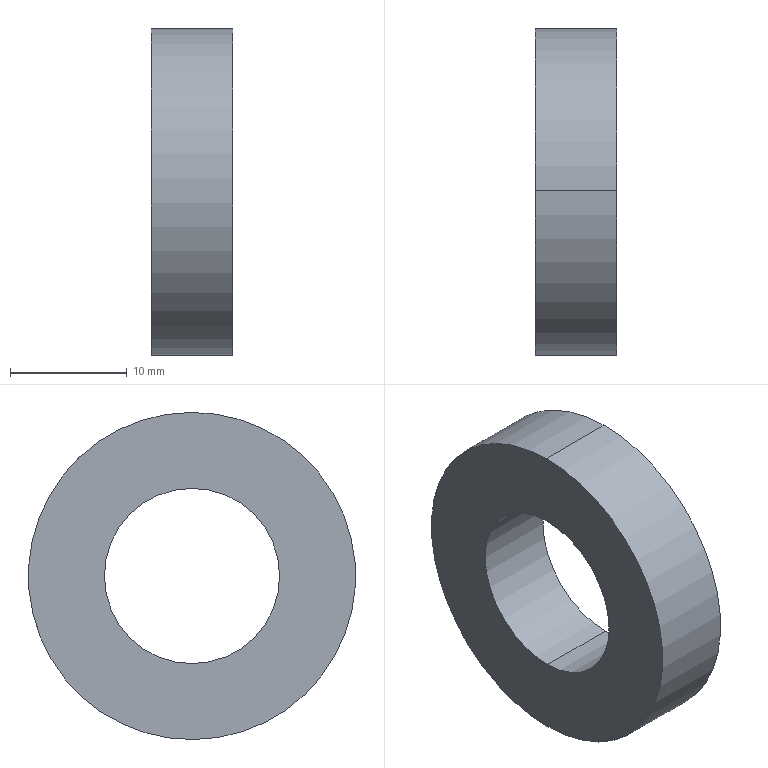Component | SolidWorks | Bearing6902-1 | 1 solid | 6 faces | box 7 x 28 x 28 mm | volume 3073 mm3 | cylinder 4 | plane 2 | commonest cylinder face diameters 15 x2 28 x2
build123d program:
from build123d import *

# Parameters (mm, degrees)
SKETCH1_R           = 14
SKETCH1_R_2         = 7.5
BOSS_EXTRUDE1_DEPTH = 7


with BuildPart() as part:
    # Sketch1 → Boss-Extrude1 (new body)
    with BuildSketch(Plane.XY):
        Circle(SKETCH1_R)
        Circle(SKETCH1_R_2, mode=Mode.SUBTRACT)
    extrude(amount=BOSS_EXTRUDE1_DEPTH)


solid = part.part

# Placed as in the assembly
solid = solid.moved(Location((1541.163, 3833.696, 1079.241), (0, 90, 0)))
STEP:
#1=CARTESIAN_POINT('',(60.951,150.935,42.785));
#2=VERTEX_POINT('',#1);
#3=CARTESIAN_POINT('',(60.951,150.931,42.195));
#4=VERTEX_POINT('',#3);
#5=CARTESIAN_POINT('',(60.951,150.933,42.49));
#6=DIRECTION('',(1.,0.0001552,0.));
#7=DIRECTION('',(0.00000119,-0.007636,-1.));
#8=AXIS2_PLACEMENT_3D('',#5,#6,#7);
#9=CIRCLE('',#8,0.2953);
#10=EDGE_CURVE('',#2,#4,#9,.T.);
#11=ORIENTED_EDGE('',*,*,#10,.T.);
#12=CARTESIAN_POINT('',(60.676,150.931,42.195));
#13=VERTEX_POINT('',#12);
#14=CARTESIAN_POINT('',(60.951,150.931,42.195));
#15=DIRECTION('',(-1.,-0.0001552,-0.));
#16=VECTOR('',#15,39.37);
#17=LINE('',#14,#16);
#18=EDGE_CURVE('',#4,#13,#17,.T.);
#19=ORIENTED_EDGE('',*,*,#18,.T.);
#20=CARTESIAN_POINT('',(60.676,150.935,42.785));
#21=VERTEX_POINT('',#20);
#22=CARTESIAN_POINT('',(60.676,150.933,42.49));
#23=DIRECTION('',(1.,0.0001552,0.));
#24=DIRECTION('',(0.00000119,-0.007636,-1.));
#25=AXIS2_PLACEMENT_3D('',#22,#23,#24);
#26=CIRCLE('',#25,0.2953);
#27=EDGE_CURVE('',#21,#13,#26,.T.);
#28=ORIENTED_EDGE('',*,*,#27,.F.);
#29=CARTESIAN_POINT('',(60.951,150.935,42.785));
#30=DIRECTION('',(-1.,-0.0001552,-0.));
#31=VECTOR('',#30,39.37);
#32=LINE('',#29,#31);
#33=EDGE_CURVE('',#2,#21,#32,.T.);
#34=ORIENTED_EDGE('',*,*,#33,.F.);
#35=EDGE_LOOP('',(#11,#19,#28,#34));
#36=FACE_OUTER_BOUND('',#35,.T.);
#37=CARTESIAN_POINT('',(60.951,150.933,42.49));
#38=DIRECTION('',(-1.,-0.0001552,-0.));
#39=DIRECTION('',(-0.00000119,0.007636,1.));
#40=AXIS2_PLACEMENT_3D('',#37,#38,#39);
#41=CYLINDRICAL_SURFACE('',#40,0.2953);
#42=ADVANCED_FACE('',(#36),#41,.F.);
#43=CARTESIAN_POINT('',(60.951,150.929,41.939));
#44=VERTEX_POINT('',#43);
#45=CARTESIAN_POINT('',(60.951,150.937,43.041));
#46=VERTEX_POINT('',#45);
#47=CARTESIAN_POINT('',(60.951,150.933,42.49));
#48=DIRECTION('',(1.,0.0001552,0.));
#49=DIRECTION('',(0.00000119,-0.007636,-1.));
#50=AXIS2_PLACEMENT_3D('',#47,#48,#49);
#51=CIRCLE('',#50,0.5512);
#52=EDGE_CURVE('',#44,#46,#51,.T.);
#53=ORIENTED_EDGE('',*,*,#52,.F.);
#54=CARTESIAN_POINT('',(60.676,150.929,41.939));
#55=VERTEX_POINT('',#54);
#56=CARTESIAN_POINT('',(60.951,150.929,41.939));
#57=DIRECTION('',(-1.,-0.0001552,-0.));
#58=VECTOR('',#57,39.37);
#59=LINE('',#56,#58);
#60=EDGE_CURVE('',#44,#55,#59,.T.);
#61=ORIENTED_EDGE('',*,*,#60,.T.);
#62=CARTESIAN_POINT('',(60.676,150.937,43.041));
#63=VERTEX_POINT('',#62);
#64=CARTESIAN_POINT('',(60.676,150.933,42.49));
#65=DIRECTION('',(1.,0.0001552,0.));
#66=DIRECTION('',(0.00000119,-0.007636,-1.));
#67=AXIS2_PLACEMENT_3D('',#64,#65,#66);
#68=CIRCLE('',#67,0.5512);
#69=EDGE_CURVE('',#55,#63,#68,.T.);
#70=ORIENTED_EDGE('',*,*,#69,.T.);
#71=CARTESIAN_POINT('',(60.951,150.937,43.041));
#72=DIRECTION('',(-1.,-0.0001552,-0.));
#73=VECTOR('',#72,39.37);
#74=LINE('',#71,#73);
#75=EDGE_CURVE('',#46,#63,#74,.T.);
#76=ORIENTED_EDGE('',*,*,#75,.F.);
#77=EDGE_LOOP('',(#53,#61,#70,#76));
#78=FACE_OUTER_BOUND('',#77,.T.);
#79=CARTESIAN_POINT('',(60.951,150.933,42.49));
#80=DIRECTION('',(-1.,-0.0001552,-0.));
#81=DIRECTION('',(-0.00000119,0.007636,1.));
#82=AXIS2_PLACEMENT_3D('',#79,#80,#81);
#83=CYLINDRICAL_SURFACE('',#82,0.5512);
#84=ADVANCED_FACE('',(#78),#83,.T.);
#85=CARTESIAN_POINT('',(60.951,150.933,42.49));
#86=DIRECTION('',(1.,0.0001552,0.));
#87=DIRECTION('',(0.00000119,-0.007636,-1.));
#88=AXIS2_PLACEMENT_3D('',#85,#86,#87);
#89=CIRCLE('',#88,0.5512);
#90=EDGE_CURVE('',#46,#44,#89,.T.);
#91=ORIENTED_EDGE('',*,*,#90,.T.);
#92=ORIENTED_EDGE('',*,*,#52,.T.);
#93=EDGE_LOOP('',(#91,#92));
#94=FACE_OUTER_BOUND('',#93,.T.);
#95=ORIENTED_EDGE('',*,*,#10,.F.);
#96=CARTESIAN_POINT('',(60.951,150.933,42.49));
#97=DIRECTION('',(1.,0.0001552,0.));
#98=DIRECTION('',(0.00000119,-0.007636,-1.));
#99=AXIS2_PLACEMENT_3D('',#96,#97,#98);
#100=CIRCLE('',#99,0.2953);
#101=EDGE_CURVE('',#4,#2,#100,.T.);
#102=ORIENTED_EDGE('',*,*,#101,.F.);
#103=EDGE_LOOP('',(#95,#102));
#104=FACE_BOUND('',#103,.T.);
#105=CARTESIAN_POINT('',(60.951,150.933,42.49));
#106=DIRECTION('',(1.,0.0001552,0.));
#107=DIRECTION('',(0.00000119,-0.007636,-1.));
#108=AXIS2_PLACEMENT_3D('',#105,#106,#107);
#109=PLANE('',#108);
#110=ADVANCED_FACE('',(#94,#104),#109,.T.);
#111=CARTESIAN_POINT('',(60.676,150.933,42.49));
#112=DIRECTION('',(1.,0.0001552,0.));
#113=DIRECTION('',(0.00000119,-0.007636,-1.));
#114=AXIS2_PLACEMENT_3D('',#111,#112,#113);
#115=CIRCLE('',#114,0.5512);
#116=EDGE_CURVE('',#63,#55,#115,.T.);
#117=ORIENTED_EDGE('',*,*,#116,.F.);
#118=ORIENTED_EDGE('',*,*,#69,.F.);
#119=EDGE_LOOP('',(#117,#118));
#120=FACE_OUTER_BOUND('',#119,.T.);
#121=ORIENTED_EDGE('',*,*,#27,.T.);
#122=CARTESIAN_POINT('',(60.676,150.933,42.49));
#123=DIRECTION('',(1.,0.0001552,0.));
#124=DIRECTION('',(0.00000119,-0.007636,-1.));
#125=AXIS2_PLACEMENT_3D('',#122,#123,#124);
#126=CIRCLE('',#125,0.2953);
#127=EDGE_CURVE('',#13,#21,#126,.T.);
#128=ORIENTED_EDGE('',*,*,#127,.T.);
#129=EDGE_LOOP('',(#121,#128));
#130=FACE_BOUND('',#129,.T.);
#131=CARTESIAN_POINT('',(60.676,150.933,42.49));
#132=DIRECTION('',(1.,0.0001552,0.));
#133=DIRECTION('',(0.00000119,-0.007636,-1.));
#134=AXIS2_PLACEMENT_3D('',#131,#132,#133);
#135=PLANE('',#134);
#136=ADVANCED_FACE('',(#120,#130),#135,.F.);
#137=ORIENTED_EDGE('',*,*,#60,.F.);
#138=ORIENTED_EDGE('',*,*,#90,.F.);
#139=ORIENTED_EDGE('',*,*,#75,.T.);
#140=ORIENTED_EDGE('',*,*,#116,.T.);
#141=EDGE_LOOP('',(#137,#138,#139,#140));
#142=FACE_OUTER_BOUND('',#141,.T.);
#143=CARTESIAN_POINT('',(60.951,150.933,42.49));
#144=DIRECTION('',(-1.,-0.0001552,-0.));
#145=DIRECTION('',(-0.00000119,0.007636,1.));
#146=AXIS2_PLACEMENT_3D('',#143,#144,#145);
#147=CYLINDRICAL_SURFACE('',#146,0.5512);
#148=ADVANCED_FACE('',(#142),#147,.T.);
#149=ORIENTED_EDGE('',*,*,#18,.F.);
#150=ORIENTED_EDGE('',*,*,#101,.T.);
#151=ORIENTED_EDGE('',*,*,#33,.T.);
#152=ORIENTED_EDGE('',*,*,#127,.F.);
#153=EDGE_LOOP('',(#149,#150,#151,#152));
#154=FACE_OUTER_BOUND('',#153,.T.);
#155=CARTESIAN_POINT('',(60.951,150.933,42.49));
#156=DIRECTION('',(-1.,-0.0001552,-0.));
#157=DIRECTION('',(-0.00000119,0.007636,1.));
#158=AXIS2_PLACEMENT_3D('',#155,#156,#157);
#159=CYLINDRICAL_SURFACE('',#158,0.2953);
#160=ADVANCED_FACE('',(#154),#159,.F.);
#161=CLOSED_SHELL('',(#42,#84,#110,#136,#148,#160));
#162=MANIFOLD_SOLID_BREP('',#161);
#163=CARTESIAN_POINT('',(0.,0.,0.));
#164=DIRECTION('',(0.,0.,1.));
#165=DIRECTION('',(1.,0.,0.));
#166=AXIS2_PLACEMENT_3D('',#163,#164,#165);
#167=(LENGTH_UNIT()NAMED_UNIT(*)SI_UNIT($,.METRE.));
#168=LENGTH_MEASURE_WITH_UNIT(LENGTH_MEASURE(0.0254),#167);
#169=DIMENSIONAL_EXPONENTS(1.,0.,0.,0.,0.,0.,0.);
#170=(CONVERSION_BASED_UNIT('',#168)LENGTH_UNIT()NAMED_UNIT(#169));
#171=UNCERTAINTY_MEASURE_WITH_UNIT(LENGTH_MEASURE(0.00001),#170,'','');
#172=(NAMED_UNIT(*)PLANE_ANGLE_UNIT()SI_UNIT($,.RADIAN.));
#173=(NAMED_UNIT(*)SI_UNIT($,.STERADIAN.)SOLID_ANGLE_UNIT());
#174=(GEOMETRIC_REPRESENTATION_CONTEXT(3)GLOBAL_UNCERTAINTY_ASSIGNED_CONTEXT((#171))GLOBAL_UNIT_ASSIGNED_CONTEXT((#170,#172,#173))REPRESENTATION_CONTEXT('',''));
#175=ADVANCED_BREP_SHAPE_REPRESENTATION('',(#162,#166),#174);
#176=COLOUR_RGB('',0.7922,0.8196,0.9333);
#177=FILL_AREA_STYLE_COLOUR('',#176);
#178=FILL_AREA_STYLE('',(#177));
#179=SURFACE_STYLE_FILL_AREA(#178);
#180=SURFACE_SIDE_STYLE('',(#179));
#181=SURFACE_STYLE_USAGE(.BOTH.,#180);
#182=PRESENTATION_STYLE_ASSIGNMENT((#181));
#183=STYLED_ITEM('',(#182),#162);
#184=PRESENTATION_LAYER_ASSIGNMENT('','',(#183));
#185=(LENGTH_UNIT()NAMED_UNIT(*)SI_UNIT($,.METRE.));
#186=LENGTH_MEASURE_WITH_UNIT(LENGTH_MEASURE(0.0254),#185);
#187=DIMENSIONAL_EXPONENTS(1.,0.,0.,0.,0.,0.,0.);
#188=(CONVERSION_BASED_UNIT('',#186)LENGTH_UNIT()NAMED_UNIT(#187));
#189=UNCERTAINTY_MEASURE_WITH_UNIT(LENGTH_MEASURE(0.00001),#188,'','');
#190=(NAMED_UNIT(*)PLANE_ANGLE_UNIT()SI_UNIT($,.RADIAN.));
#191=(NAMED_UNIT(*)SI_UNIT($,.STERADIAN.)SOLID_ANGLE_UNIT());
#192=(GEOMETRIC_REPRESENTATION_CONTEXT(3)GLOBAL_UNCERTAINTY_ASSIGNED_CONTEXT((#189))GLOBAL_UNIT_ASSIGNED_CONTEXT((#188,#190,#191))REPRESENTATION_CONTEXT('',''));
#193=MECHANICAL_DESIGN_GEOMETRIC_PRESENTATION_REPRESENTATION('',(#183),#192);